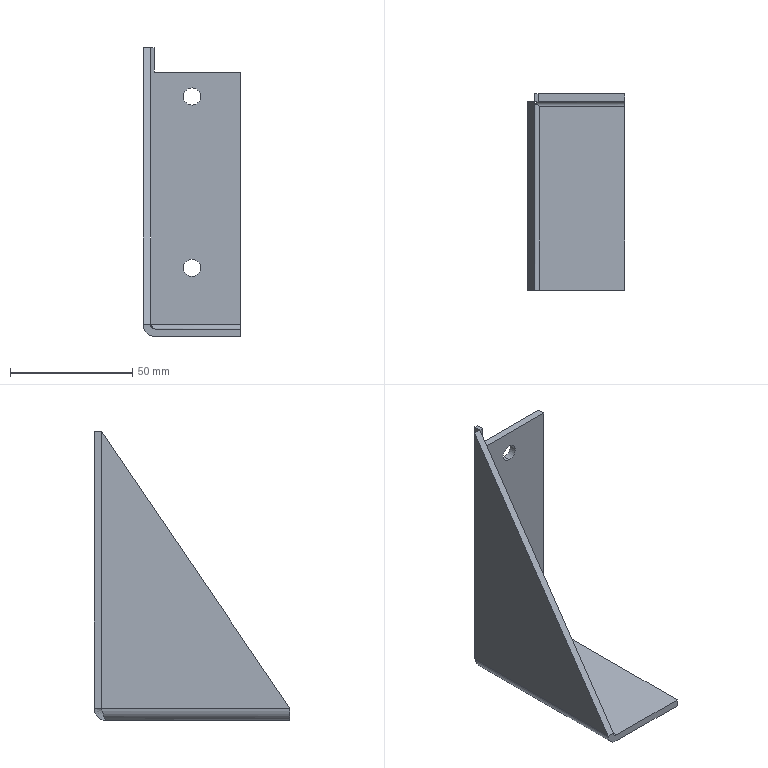Component | SolidWorks | ButtonStation-1_BracketAssembly-1_Bracket4-1 | 1 solid | 24 faces | box 40 x 80 x 118 mm | volume 33984 mm3 | plane 14 | cylinder 8 | spline 2 | commonest cylinder face diameters 7 x4 4 x2 10 x2 | material Plain Carbon Steel
STEP:
#1=COLOUR_RGB('',0.7922,0.8196,0.9333);
#2=FILL_AREA_STYLE_COLOUR('',#1);
#3=FILL_AREA_STYLE('',(#2));
#4=SURFACE_STYLE_FILL_AREA(#3);
#5=SURFACE_SIDE_STYLE('',(#4));
#6=SURFACE_STYLE_USAGE(.BOTH.,#5);
#7=PRESENTATION_STYLE_ASSIGNMENT((#6));
#8=CARTESIAN_POINT('',(-9.449,24.685,25.846));
#9=VERTEX_POINT('',#8);
#10=CARTESIAN_POINT('',(-9.449,24.685,25.571));
#11=VERTEX_POINT('',#10);
#12=CARTESIAN_POINT('',(-9.449,24.685,25.709));
#13=DIRECTION('',(0.,-1.,0.));
#14=DIRECTION('',(0.,0.,1.));
#15=AXIS2_PLACEMENT_3D('',#12,#13,#14);
#16=CIRCLE('',#15,0.1378);
#17=EDGE_CURVE('',#9,#11,#16,.T.);
#18=ORIENTED_EDGE('',*,*,#17,.T.);
#19=CARTESIAN_POINT('',(-9.449,24.803,25.571));
#20=VERTEX_POINT('',#19);
#21=CARTESIAN_POINT('',(-9.449,24.685,25.571));
#22=DIRECTION('',(0.,1.,-0.));
#23=VECTOR('',#22,39.37);
#24=LINE('',#21,#23);
#25=EDGE_CURVE('',#11,#20,#24,.T.);
#26=ORIENTED_EDGE('',*,*,#25,.T.);
#27=CARTESIAN_POINT('',(-9.449,24.803,25.846));
#28=VERTEX_POINT('',#27);
#29=CARTESIAN_POINT('',(-9.449,24.803,25.709));
#30=DIRECTION('',(0.,-1.,0.));
#31=DIRECTION('',(0.,0.,1.));
#32=AXIS2_PLACEMENT_3D('',#29,#30,#31);
#33=CIRCLE('',#32,0.1378);
#34=EDGE_CURVE('',#28,#20,#33,.T.);
#35=ORIENTED_EDGE('',*,*,#34,.F.);
#36=CARTESIAN_POINT('',(-9.449,24.685,25.846));
#37=DIRECTION('',(0.,1.,-0.));
#38=VECTOR('',#37,39.37);
#39=LINE('',#36,#38);
#40=EDGE_CURVE('',#9,#28,#39,.T.);
#41=ORIENTED_EDGE('',*,*,#40,.F.);
#42=EDGE_LOOP('',(#18,#26,#35,#41));
#43=FACE_OUTER_BOUND('',#42,.T.);
#44=CARTESIAN_POINT('',(-9.449,24.685,25.709));
#45=DIRECTION('',(0.,1.,-0.));
#46=DIRECTION('',(0.,0.,1.));
#47=AXIS2_PLACEMENT_3D('',#44,#45,#46);
#48=CYLINDRICAL_SURFACE('',#47,0.1378);
#49=ADVANCED_FACE('',(#43),#48,.F.);
#50=CARTESIAN_POINT('',(-9.449,24.685,23.091));
#51=VERTEX_POINT('',#50);
#52=CARTESIAN_POINT('',(-9.449,24.685,22.815));
#53=VERTEX_POINT('',#52);
#54=CARTESIAN_POINT('',(-9.449,24.685,22.953));
#55=DIRECTION('',(0.,-1.,0.));
#56=DIRECTION('',(0.,0.,1.));
#57=AXIS2_PLACEMENT_3D('',#54,#55,#56);
#58=CIRCLE('',#57,0.1378);
#59=EDGE_CURVE('',#51,#53,#58,.T.);
#60=ORIENTED_EDGE('',*,*,#59,.T.);
#61=CARTESIAN_POINT('',(-9.449,24.803,22.815));
#62=VERTEX_POINT('',#61);
#63=CARTESIAN_POINT('',(-9.449,24.685,22.815));
#64=DIRECTION('',(0.,1.,-0.));
#65=VECTOR('',#64,39.37);
#66=LINE('',#63,#65);
#67=EDGE_CURVE('',#53,#62,#66,.T.);
#68=ORIENTED_EDGE('',*,*,#67,.T.);
#69=CARTESIAN_POINT('',(-9.449,24.803,23.091));
#70=VERTEX_POINT('',#69);
#71=CARTESIAN_POINT('',(-9.449,24.803,22.953));
#72=DIRECTION('',(0.,-1.,0.));
#73=DIRECTION('',(0.,0.,1.));
#74=AXIS2_PLACEMENT_3D('',#71,#72,#73);
#75=CIRCLE('',#74,0.1378);
#76=EDGE_CURVE('',#70,#62,#75,.T.);
#77=ORIENTED_EDGE('',*,*,#76,.F.);
#78=CARTESIAN_POINT('',(-9.449,24.685,23.091));
#79=DIRECTION('',(0.,1.,-0.));
#80=VECTOR('',#79,39.37);
#81=LINE('',#78,#80);
#82=EDGE_CURVE('',#51,#70,#81,.T.);
#83=ORIENTED_EDGE('',*,*,#82,.F.);
#84=EDGE_LOOP('',(#60,#68,#77,#83));
#85=FACE_OUTER_BOUND('',#84,.T.);
#86=CARTESIAN_POINT('',(-9.449,24.685,22.953));
#87=DIRECTION('',(0.,1.,-0.));
#88=DIRECTION('',(0.,0.,1.));
#89=AXIS2_PLACEMENT_3D('',#86,#87,#88);
#90=CYLINDRICAL_SURFACE('',#89,0.1378);
#91=ADVANCED_FACE('',(#85),#90,.F.);
#92=CARTESIAN_POINT('',(-10.118,24.682,22.047));
#93=VERTEX_POINT('',#92);
#94=CARTESIAN_POINT('',(-10.118,21.654,22.047));
#95=VERTEX_POINT('',#94);
#96=CARTESIAN_POINT('',(-10.118,21.654,22.047));
#97=DIRECTION('',(0.,-1.,0.));
#98=VECTOR('',#97,39.37);
#99=LINE('',#96,#98);
#100=EDGE_CURVE('',#93,#95,#99,.T.);
#101=ORIENTED_EDGE('',*,*,#100,.F.);
#102=CARTESIAN_POINT('',(-10.118,24.682,26.496));
#103=VERTEX_POINT('',#102);
#104=CARTESIAN_POINT('',(-10.118,24.682,21.969));
#105=DIRECTION('',(0.,0.,-1.));
#106=VECTOR('',#105,39.37);
#107=LINE('',#104,#106);
#108=EDGE_CURVE('',#103,#93,#107,.T.);
#109=ORIENTED_EDGE('',*,*,#108,.F.);
#110=CARTESIAN_POINT('',(-10.118,21.654,22.047));
#111=DIRECTION('',(-0.,0.5628,0.8266));
#112=VECTOR('',#111,39.37);
#113=LINE('',#110,#112);
#114=EDGE_CURVE('',#95,#103,#113,.T.);
#115=ORIENTED_EDGE('',*,*,#114,.F.);
#116=EDGE_LOOP('',(#101,#109,#115));
#117=FACE_OUTER_BOUND('',#116,.T.);
#118=CARTESIAN_POINT('',(-10.118,21.654,21.969));
#119=DIRECTION('',(-1.,0.,-0.));
#120=DIRECTION('',(-0.,0.,1.));
#121=AXIS2_PLACEMENT_3D('',#118,#119,#120);
#122=PLANE('',#121);
#123=ADVANCED_FACE('',(#117),#122,.F.);
#124=CARTESIAN_POINT('',(-10.236,21.654,22.047));
#125=VERTEX_POINT('',#124);
#126=CARTESIAN_POINT('',(-10.236,21.654,22.047));
#127=DIRECTION('',(-1.,0.,-0.));
#128=VECTOR('',#127,39.37);
#129=LINE('',#126,#128);
#130=EDGE_CURVE('',#95,#125,#129,.T.);
#131=ORIENTED_EDGE('',*,*,#130,.F.);
#132=ORIENTED_EDGE('',*,*,#114,.T.);
#133=CARTESIAN_POINT('',(-10.236,24.682,26.496));
#134=VERTEX_POINT('',#133);
#135=CARTESIAN_POINT('',(-10.236,24.682,26.496));
#136=DIRECTION('',(1.,-0.,0.));
#137=VECTOR('',#136,39.37);
#138=LINE('',#135,#137);
#139=EDGE_CURVE('',#134,#103,#138,.T.);
#140=ORIENTED_EDGE('',*,*,#139,.F.);
#141=CARTESIAN_POINT('',(-10.236,24.682,26.496));
#142=DIRECTION('',(0.,0.5628,0.8266));
#143=VECTOR('',#142,39.37);
#144=LINE('',#141,#143);
#145=EDGE_CURVE('',#125,#134,#144,.T.);
#146=ORIENTED_EDGE('',*,*,#145,.F.);
#147=EDGE_LOOP('',(#131,#132,#140,#146));
#148=FACE_OUTER_BOUND('',#147,.T.);
#149=CARTESIAN_POINT('',(-10.236,24.682,26.496));
#150=DIRECTION('',(0.,0.8266,-0.5628));
#151=DIRECTION('',(0.,0.5628,0.8266));
#152=AXIS2_PLACEMENT_3D('',#149,#150,#151);
#153=PLANE('',#152);
#154=ADVANCED_FACE('',(#148),#153,.F.);
#155=CARTESIAN_POINT('',(-10.039,24.606,21.969));
#156=VERTEX_POINT('',#155);
#157=CARTESIAN_POINT('',(-10.118,24.682,22.047));
#158=CARTESIAN_POINT('',(-10.118,24.676,22.037));
#159=CARTESIAN_POINT('',(-10.116,24.67,22.027));
#160=CARTESIAN_POINT('',(-10.11,24.66,22.012));
#161=CARTESIAN_POINT('',(-10.108,24.657,22.008));
#162=CARTESIAN_POINT('',(-10.102,24.651,21.999));
#163=CARTESIAN_POINT('',(-10.099,24.648,21.995));
#164=CARTESIAN_POINT('',(-10.091,24.641,21.988));
#165=CARTESIAN_POINT('',(-10.087,24.638,21.985));
#166=CARTESIAN_POINT('',(-10.079,24.632,21.979));
#167=CARTESIAN_POINT('',(-10.074,24.629,21.977));
#168=CARTESIAN_POINT('',(-10.065,24.622,21.973));
#169=CARTESIAN_POINT('',(-10.06,24.619,21.971));
#170=CARTESIAN_POINT('',(-10.05,24.613,21.969));
#171=CARTESIAN_POINT('',(-10.045,24.609,21.969));
#172=CARTESIAN_POINT('',(-10.039,24.606,21.969));
#173=B_SPLINE_CURVE_WITH_KNOTS('',3,(#157,#158,#159,#160,#161,#162,#163,#164,#165,#166,#167,#168,#169,#170,#171,#172),.UNSPECIFIED.,.F.,.F.,(4,2,2,2,2,2,2,4),(0.,0.0009146,0.001372,0.001829,0.002286,0.002744,0.003201,0.003658),.UNSPECIFIED.);
#174=EDGE_CURVE('',#93,#156,#173,.T.);
#175=ORIENTED_EDGE('',*,*,#174,.F.);
#176=ORIENTED_EDGE('',*,*,#100,.T.);
#177=CARTESIAN_POINT('',(-10.039,21.654,21.969));
#178=VERTEX_POINT('',#177);
#179=CARTESIAN_POINT('',(-10.039,21.654,22.047));
#180=DIRECTION('',(0.,1.,0.));
#181=DIRECTION('',(0.,0.,-1.));
#182=AXIS2_PLACEMENT_3D('',#179,#180,#181);
#183=CIRCLE('',#182,0.07874);
#184=EDGE_CURVE('',#178,#95,#183,.T.);
#185=ORIENTED_EDGE('',*,*,#184,.F.);
#186=CARTESIAN_POINT('',(-10.039,21.654,21.969));
#187=DIRECTION('',(0.,-1.,0.));
#188=VECTOR('',#187,39.37);
#189=LINE('',#186,#188);
#190=EDGE_CURVE('',#156,#178,#189,.T.);
#191=ORIENTED_EDGE('',*,*,#190,.F.);
#192=EDGE_LOOP('',(#175,#176,#185,#191));
#193=FACE_OUTER_BOUND('',#192,.T.);
#194=CARTESIAN_POINT('',(-10.039,21.654,22.047));
#195=DIRECTION('',(0.,-1.,0.));
#196=DIRECTION('',(0.,0.,-1.));
#197=AXIS2_PLACEMENT_3D('',#194,#195,#196);
#198=CYLINDRICAL_SURFACE('',#197,0.07874);
#199=ADVANCED_FACE('',(#193),#198,.F.);
#200=CARTESIAN_POINT('',(-10.236,24.682,22.047));
#201=VERTEX_POINT('',#200);
#202=CARTESIAN_POINT('',(-10.118,24.682,22.047));
#203=DIRECTION('',(-1.,0.,0.));
#204=VECTOR('',#203,39.37);
#205=LINE('',#202,#204);
#206=EDGE_CURVE('',#93,#201,#205,.T.);
#207=ORIENTED_EDGE('',*,*,#206,.T.);
#208=CARTESIAN_POINT('',(-10.236,24.682,21.969));
#209=DIRECTION('',(0.,0.,1.));
#210=VECTOR('',#209,39.37);
#211=LINE('',#208,#210);
#212=EDGE_CURVE('',#201,#134,#211,.T.);
#213=ORIENTED_EDGE('',*,*,#212,.T.);
#214=ORIENTED_EDGE('',*,*,#139,.T.);
#215=ORIENTED_EDGE('',*,*,#108,.T.);
#216=EDGE_LOOP('',(#207,#213,#214,#215));
#217=FACE_OUTER_BOUND('',#216,.T.);
#218=CARTESIAN_POINT('',(-10.118,24.682,21.969));
#219=DIRECTION('',(0.,1.,0.));
#220=DIRECTION('',(0.,0.,1.));
#221=AXIS2_PLACEMENT_3D('',#218,#219,#220);
#222=PLANE('',#221);
#223=ADVANCED_FACE('',(#217),#222,.T.);
#224=ORIENTED_EDGE('',*,*,#145,.T.);
#225=ORIENTED_EDGE('',*,*,#212,.F.);
#226=CARTESIAN_POINT('',(-10.236,21.654,22.047));
#227=DIRECTION('',(0.,-1.,0.));
#228=VECTOR('',#227,39.37);
#229=LINE('',#226,#228);
#230=EDGE_CURVE('',#201,#125,#229,.T.);
#231=ORIENTED_EDGE('',*,*,#230,.T.);
#232=EDGE_LOOP('',(#224,#225,#231));
#233=FACE_OUTER_BOUND('',#232,.T.);
#234=CARTESIAN_POINT('',(-10.236,21.654,21.969));
#235=DIRECTION('',(-1.,0.,-0.));
#236=DIRECTION('',(-0.,0.,1.));
#237=AXIS2_PLACEMENT_3D('',#234,#235,#236);
#238=PLANE('',#237);
#239=ADVANCED_FACE('',(#233),#238,.T.);
#240=ORIENTED_EDGE('',*,*,#130,.T.);
#241=CARTESIAN_POINT('',(-10.039,21.654,21.85));
#242=VERTEX_POINT('',#241);
#243=CARTESIAN_POINT('',(-10.039,21.654,22.047));
#244=DIRECTION('',(0.,1.,0.));
#245=DIRECTION('',(0.,0.,-1.));
#246=AXIS2_PLACEMENT_3D('',#243,#244,#245);
#247=CIRCLE('',#246,0.1969);
#248=EDGE_CURVE('',#242,#125,#247,.T.);
#249=ORIENTED_EDGE('',*,*,#248,.F.);
#250=CARTESIAN_POINT('',(-8.661,21.654,21.85));
#251=VERTEX_POINT('',#250);
#252=CARTESIAN_POINT('',(-10.118,21.654,21.85));
#253=DIRECTION('',(-1.,0.,0.));
#254=VECTOR('',#253,39.37);
#255=LINE('',#252,#254);
#256=EDGE_CURVE('',#251,#242,#255,.T.);
#257=ORIENTED_EDGE('',*,*,#256,.F.);
#258=CARTESIAN_POINT('',(-8.661,21.654,21.969));
#259=VERTEX_POINT('',#258);
#260=CARTESIAN_POINT('',(-8.661,21.654,21.969));
#261=DIRECTION('',(0.,0.,-1.));
#262=VECTOR('',#261,39.37);
#263=LINE('',#260,#262);
#264=EDGE_CURVE('',#259,#251,#263,.T.);
#265=ORIENTED_EDGE('',*,*,#264,.F.);
#266=CARTESIAN_POINT('',(-10.118,21.654,21.969));
#267=DIRECTION('',(-1.,0.,0.));
#268=VECTOR('',#267,39.37);
#269=LINE('',#266,#268);
#270=EDGE_CURVE('',#259,#178,#269,.T.);
#271=ORIENTED_EDGE('',*,*,#270,.T.);
#272=ORIENTED_EDGE('',*,*,#184,.T.);
#273=EDGE_LOOP('',(#240,#249,#257,#265,#271,#272));
#274=FACE_OUTER_BOUND('',#273,.T.);
#275=CARTESIAN_POINT('',(-10.039,21.654,22.047));
#276=DIRECTION('',(0.,1.,0.));
#277=DIRECTION('',(0.,0.,1.));
#278=AXIS2_PLACEMENT_3D('',#275,#276,#277);
#279=PLANE('',#278);
#280=ADVANCED_FACE('',(#274),#279,.F.);
#281=ORIENTED_EDGE('',*,*,#190,.T.);
#282=ORIENTED_EDGE('',*,*,#270,.F.);
#283=CARTESIAN_POINT('',(-8.661,24.606,21.969));
#284=VERTEX_POINT('',#283);
#285=CARTESIAN_POINT('',(-8.661,24.685,21.969));
#286=DIRECTION('',(0.,-1.,0.));
#287=VECTOR('',#286,39.37);
#288=LINE('',#285,#287);
#289=EDGE_CURVE('',#284,#259,#288,.T.);
#290=ORIENTED_EDGE('',*,*,#289,.F.);
#291=CARTESIAN_POINT('',(-10.118,24.606,21.969));
#292=DIRECTION('',(1.,0.,0.));
#293=VECTOR('',#292,39.37);
#294=LINE('',#291,#293);
#295=EDGE_CURVE('',#156,#284,#294,.T.);
#296=ORIENTED_EDGE('',*,*,#295,.F.);
#297=EDGE_LOOP('',(#281,#282,#290,#296));
#298=FACE_OUTER_BOUND('',#297,.T.);
#299=CARTESIAN_POINT('',(-10.118,24.685,21.969));
#300=DIRECTION('',(0.,0.,-1.));
#301=DIRECTION('',(-1.,0.,0.));
#302=AXIS2_PLACEMENT_3D('',#299,#300,#301);
#303=PLANE('',#302);
#304=ADVANCED_FACE('',(#298),#303,.F.);
#305=ORIENTED_EDGE('',*,*,#174,.T.);
#306=CARTESIAN_POINT('',(-10.039,24.606,21.85));
#307=VERTEX_POINT('',#306);
#308=CARTESIAN_POINT('',(-10.039,24.606,21.909));
#309=DIRECTION('',(0.,0.,1.));
#310=VECTOR('',#309,39.37);
#311=LINE('',#308,#310);
#312=EDGE_CURVE('',#307,#156,#311,.T.);
#313=ORIENTED_EDGE('',*,*,#312,.F.);
#314=CARTESIAN_POINT('',(-10.236,24.682,22.047));
#315=CARTESIAN_POINT('',(-10.236,24.679,22.034));
#316=CARTESIAN_POINT('',(-10.235,24.676,22.021));
#317=CARTESIAN_POINT('',(-10.23,24.67,21.996));
#318=CARTESIAN_POINT('',(-10.226,24.666,21.984));
#319=CARTESIAN_POINT('',(-10.216,24.66,21.96));
#320=CARTESIAN_POINT('',(-10.21,24.657,21.949));
#321=CARTESIAN_POINT('',(-10.196,24.651,21.927));
#322=CARTESIAN_POINT('',(-10.188,24.647,21.917));
#323=CARTESIAN_POINT('',(-10.17,24.641,21.899));
#324=CARTESIAN_POINT('',(-10.16,24.638,21.891));
#325=CARTESIAN_POINT('',(-10.138,24.632,21.876));
#326=CARTESIAN_POINT('',(-10.127,24.628,21.87));
#327=CARTESIAN_POINT('',(-10.103,24.622,21.861));
#328=CARTESIAN_POINT('',(-10.091,24.619,21.857));
#329=CARTESIAN_POINT('',(-10.065,24.613,21.852));
#330=CARTESIAN_POINT('',(-10.052,24.609,21.85));
#331=CARTESIAN_POINT('',(-10.039,24.606,21.85));
#332=B_SPLINE_CURVE_WITH_KNOTS('',3,(#314,#315,#316,#317,#318,#319,#320,#321,#322,#323,#324,#325,#326,#327,#328,#329,#330,#331),.UNSPECIFIED.,.F.,.F.,(4,2,2,2,2,2,2,2,4),(0.,0.001008,0.002017,0.003025,0.004033,0.005041,0.00605,0.007058,0.008066),.UNSPECIFIED.);
#333=EDGE_CURVE('',#201,#307,#332,.T.);
#334=ORIENTED_EDGE('',*,*,#333,.F.);
#335=ORIENTED_EDGE('',*,*,#206,.F.);
#336=EDGE_LOOP('',(#305,#313,#334,#335));
#337=FACE_OUTER_BOUND('',#336,.T.);
#338=CARTESIAN_POINT('',(-10.039,24.606,21.849));
#339=CARTESIAN_POINT('',(-10.065,24.613,21.849));
#340=CARTESIAN_POINT('',(-10.091,24.619,21.854));
#341=CARTESIAN_POINT('',(-10.139,24.632,21.874));
#342=CARTESIAN_POINT('',(-10.161,24.638,21.889));
#343=CARTESIAN_POINT('',(-10.198,24.651,21.926));
#344=CARTESIAN_POINT('',(-10.212,24.657,21.948));
#345=CARTESIAN_POINT('',(-10.232,24.67,21.995));
#346=CARTESIAN_POINT('',(-10.237,24.676,22.021));
#347=CARTESIAN_POINT('',(-10.237,24.682,22.047));
#348=CARTESIAN_POINT('',(-10.039,24.606,21.85));
#349=CARTESIAN_POINT('',(-10.065,24.613,21.85));
#350=CARTESIAN_POINT('',(-10.091,24.619,21.856));
#351=CARTESIAN_POINT('',(-10.139,24.632,21.875));
#352=CARTESIAN_POINT('',(-10.16,24.638,21.89));
#353=CARTESIAN_POINT('',(-10.197,24.651,21.926));
#354=CARTESIAN_POINT('',(-10.211,24.657,21.948));
#355=CARTESIAN_POINT('',(-10.231,24.67,21.996));
#356=CARTESIAN_POINT('',(-10.236,24.676,22.021));
#357=CARTESIAN_POINT('',(-10.236,24.682,22.047));
#358=CARTESIAN_POINT('',(-10.039,24.606,21.969));
#359=CARTESIAN_POINT('',(-10.05,24.613,21.969));
#360=CARTESIAN_POINT('',(-10.06,24.619,21.971));
#361=CARTESIAN_POINT('',(-10.079,24.632,21.978));
#362=CARTESIAN_POINT('',(-10.088,24.638,21.984));
#363=CARTESIAN_POINT('',(-10.102,24.651,21.999));
#364=CARTESIAN_POINT('',(-10.108,24.657,22.008));
#365=CARTESIAN_POINT('',(-10.116,24.67,22.027));
#366=CARTESIAN_POINT('',(-10.118,24.676,22.037));
#367=CARTESIAN_POINT('',(-10.118,24.682,22.047));
#368=CARTESIAN_POINT('',(-10.039,24.606,21.97));
#369=CARTESIAN_POINT('',(-10.05,24.613,21.97));
#370=CARTESIAN_POINT('',(-10.06,24.619,21.972));
#371=CARTESIAN_POINT('',(-10.078,24.632,21.979));
#372=CARTESIAN_POINT('',(-10.087,24.638,21.985));
#373=CARTESIAN_POINT('',(-10.101,24.651,22.));
#374=CARTESIAN_POINT('',(-10.107,24.657,22.008));
#375=CARTESIAN_POINT('',(-10.115,24.67,22.027));
#376=CARTESIAN_POINT('',(-10.117,24.676,22.037));
#377=CARTESIAN_POINT('',(-10.117,24.682,22.047));
#378=B_SPLINE_SURFACE_WITH_KNOTS('',1,3,((#338,#339,#340,#341,#342,#343,#344,#345,#346,#347),(#348,#349,#350,#351,#352,#353,#354,#355,#356,#357),(#358,#359,#360,#361,#362,#363,#364,#365,#366,#367),(#368,#369,#370,#371,#372,#373,#374,#375,#376,#377)),.UNSPECIFIED.,.F.,.F.,.F.,(2,1,1,2),(4,2,2,2,4),(-0.01,0.,1.,1.01),(0.,0.25,0.5,0.75,1.),.UNSPECIFIED.);
#379=ADVANCED_FACE('',(#337),#378,.F.);
#380=ORIENTED_EDGE('',*,*,#230,.F.);
#381=ORIENTED_EDGE('',*,*,#333,.T.);
#382=CARTESIAN_POINT('',(-10.039,21.654,21.85));
#383=DIRECTION('',(0.,-1.,0.));
#384=VECTOR('',#383,39.37);
#385=LINE('',#382,#384);
#386=EDGE_CURVE('',#307,#242,#385,.T.);
#387=ORIENTED_EDGE('',*,*,#386,.T.);
#388=ORIENTED_EDGE('',*,*,#248,.T.);
#389=EDGE_LOOP('',(#380,#381,#387,#388));
#390=FACE_OUTER_BOUND('',#389,.T.);
#391=CARTESIAN_POINT('',(-10.039,21.654,22.047));
#392=DIRECTION('',(0.,-1.,0.));
#393=DIRECTION('',(0.,0.,-1.));
#394=AXIS2_PLACEMENT_3D('',#391,#392,#393);
#395=CYLINDRICAL_SURFACE('',#394,0.1969);
#396=ADVANCED_FACE('',(#390),#395,.T.);
#397=CARTESIAN_POINT('',(-8.661,24.685,22.047));
#398=VERTEX_POINT('',#397);
#399=CARTESIAN_POINT('',(-8.661,24.606,22.047));
#400=DIRECTION('',(-1.,0.,0.));
#401=DIRECTION('',(0.,0.,1.));
#402=AXIS2_PLACEMENT_3D('',#399,#400,#401);
#403=CIRCLE('',#402,0.07874);
#404=EDGE_CURVE('',#398,#284,#403,.T.);
#405=ORIENTED_EDGE('',*,*,#404,.F.);
#406=CARTESIAN_POINT('',(-10.115,24.685,22.047));
#407=VERTEX_POINT('',#406);
#408=CARTESIAN_POINT('',(-10.115,24.685,22.047));
#409=DIRECTION('',(1.,0.,0.));
#410=VECTOR('',#409,39.37);
#411=LINE('',#408,#410);
#412=EDGE_CURVE('',#407,#398,#411,.T.);
#413=ORIENTED_EDGE('',*,*,#412,.F.);
#414=CARTESIAN_POINT('',(-10.039,24.606,21.969));
#415=CARTESIAN_POINT('',(-10.046,24.617,21.969));
#416=CARTESIAN_POINT('',(-10.052,24.627,21.971));
#417=CARTESIAN_POINT('',(-10.061,24.641,21.976));
#418=CARTESIAN_POINT('',(-10.065,24.646,21.979));
#419=CARTESIAN_POINT('',(-10.071,24.654,21.985));
#420=CARTESIAN_POINT('',(-10.074,24.658,21.988));
#421=CARTESIAN_POINT('',(-10.08,24.666,21.995));
#422=CARTESIAN_POINT('',(-10.084,24.669,21.999));
#423=CARTESIAN_POINT('',(-10.09,24.675,22.008));
#424=CARTESIAN_POINT('',(-10.093,24.677,22.012));
#425=CARTESIAN_POINT('',(-10.099,24.681,22.022));
#426=CARTESIAN_POINT('',(-10.103,24.683,22.027));
#427=CARTESIAN_POINT('',(-10.109,24.685,22.037));
#428=CARTESIAN_POINT('',(-10.112,24.685,22.042));
#429=CARTESIAN_POINT('',(-10.115,24.685,22.047));
#430=B_SPLINE_CURVE_WITH_KNOTS('',3,(#414,#415,#416,#417,#418,#419,#420,#421,#422,#423,#424,#425,#426,#427,#428,#429),.UNSPECIFIED.,.F.,.F.,(4,2,2,2,2,2,2,4),(0.,0.0009146,0.001372,0.001829,0.002286,0.002744,0.003201,0.003658),.UNSPECIFIED.);
#431=EDGE_CURVE('',#156,#407,#430,.T.);
#432=ORIENTED_EDGE('',*,*,#431,.F.);
#433=ORIENTED_EDGE('',*,*,#295,.T.);
#434=EDGE_LOOP('',(#405,#413,#432,#433));
#435=FACE_OUTER_BOUND('',#434,.T.);
#436=CARTESIAN_POINT('',(-10.115,24.606,22.047));
#437=DIRECTION('',(-1.,0.,0.));
#438=DIRECTION('',(0.,0.,1.));
#439=AXIS2_PLACEMENT_3D('',#436,#437,#438);
#440=CYLINDRICAL_SURFACE('',#439,0.07874);
#441=ADVANCED_FACE('',(#435),#440,.F.);
#442=CARTESIAN_POINT('',(-8.661,24.803,22.047));
#443=VERTEX_POINT('',#442);
#444=CARTESIAN_POINT('',(-8.661,24.803,26.102));
#445=VERTEX_POINT('',#444);
#446=CARTESIAN_POINT('',(-8.661,24.803,26.496));
#447=DIRECTION('',(0.,0.,1.));
#448=VECTOR('',#447,39.37);
#449=LINE('',#446,#448);
#450=EDGE_CURVE('',#443,#445,#449,.T.);
#451=ORIENTED_EDGE('',*,*,#450,.T.);
#452=CARTESIAN_POINT('',(-8.661,24.685,26.102));
#453=VERTEX_POINT('',#452);
#454=CARTESIAN_POINT('',(-8.661,21.654,26.102));
#455=DIRECTION('',(0.,-1.,0.));
#456=VECTOR('',#455,39.37);
#457=LINE('',#454,#456);
#458=EDGE_CURVE('',#445,#453,#457,.T.);
#459=ORIENTED_EDGE('',*,*,#458,.T.);
#460=CARTESIAN_POINT('',(-8.661,24.685,21.969));
#461=DIRECTION('',(0.,-0.,-1.));
#462=VECTOR('',#461,39.37);
#463=LINE('',#460,#462);
#464=EDGE_CURVE('',#453,#398,#463,.T.);
#465=ORIENTED_EDGE('',*,*,#464,.T.);
#466=ORIENTED_EDGE('',*,*,#404,.T.);
#467=ORIENTED_EDGE('',*,*,#289,.T.);
#468=ORIENTED_EDGE('',*,*,#264,.T.);
#469=CARTESIAN_POINT('',(-8.661,24.606,21.85));
#470=VERTEX_POINT('',#469);
#471=CARTESIAN_POINT('',(-8.661,21.654,21.85));
#472=DIRECTION('',(0.,-1.,0.));
#473=VECTOR('',#472,39.37);
#474=LINE('',#471,#473);
#475=EDGE_CURVE('',#470,#251,#474,.T.);
#476=ORIENTED_EDGE('',*,*,#475,.F.);
#477=CARTESIAN_POINT('',(-8.661,24.606,22.047));
#478=DIRECTION('',(1.,0.,0.));
#479=DIRECTION('',(0.,0.,1.));
#480=AXIS2_PLACEMENT_3D('',#477,#478,#479);
#481=CIRCLE('',#480,0.1969);
#482=EDGE_CURVE('',#470,#443,#481,.T.);
#483=ORIENTED_EDGE('',*,*,#482,.T.);
#484=EDGE_LOOP('',(#451,#459,#465,#466,#467,#468,#476,#483));
#485=FACE_OUTER_BOUND('',#484,.T.);
#486=CARTESIAN_POINT('',(-8.661,21.654,21.969));
#487=DIRECTION('',(-1.,0.,0.));
#488=DIRECTION('',(0.,0.,1.));
#489=AXIS2_PLACEMENT_3D('',#486,#487,#488);
#490=PLANE('',#489);
#491=ADVANCED_FACE('',(#485),#490,.F.);
#492=CARTESIAN_POINT('',(-10.115,24.803,22.047));
#493=VERTEX_POINT('',#492);
#494=CARTESIAN_POINT('',(-10.115,24.744,22.047));
#495=DIRECTION('',(0.,-1.,0.));
#496=VECTOR('',#495,39.37);
#497=LINE('',#494,#496);
#498=EDGE_CURVE('',#493,#407,#497,.T.);
#499=ORIENTED_EDGE('',*,*,#498,.F.);
#500=CARTESIAN_POINT('',(-10.039,24.606,21.85));
#501=CARTESIAN_POINT('',(-10.043,24.619,21.85));
#502=CARTESIAN_POINT('',(-10.046,24.632,21.852));
#503=CARTESIAN_POINT('',(-10.052,24.657,21.857));
#504=CARTESIAN_POINT('',(-10.055,24.67,21.86));
#505=CARTESIAN_POINT('',(-10.062,24.694,21.87));
#506=CARTESIAN_POINT('',(-10.065,24.705,21.876));
#507=CARTESIAN_POINT('',(-10.071,24.726,21.891));
#508=CARTESIAN_POINT('',(-10.074,24.736,21.899));
#509=CARTESIAN_POINT('',(-10.08,24.755,21.917));
#510=CARTESIAN_POINT('',(-10.084,24.763,21.927));
#511=CARTESIAN_POINT('',(-10.09,24.777,21.949));
#512=CARTESIAN_POINT('',(-10.093,24.783,21.96));
#513=CARTESIAN_POINT('',(-10.099,24.793,21.984));
#514=CARTESIAN_POINT('',(-10.103,24.797,21.996));
#515=CARTESIAN_POINT('',(-10.109,24.802,22.021));
#516=CARTESIAN_POINT('',(-10.112,24.803,22.034));
#517=CARTESIAN_POINT('',(-10.115,24.803,22.047));
#518=B_SPLINE_CURVE_WITH_KNOTS('',3,(#500,#501,#502,#503,#504,#505,#506,#507,#508,#509,#510,#511,#512,#513,#514,#515,#516,#517),.UNSPECIFIED.,.F.,.F.,(4,2,2,2,2,2,2,2,4),(0.,0.001008,0.002017,0.003025,0.004033,0.005041,0.00605,0.007058,0.008066),.UNSPECIFIED.);
#519=EDGE_CURVE('',#307,#493,#518,.T.);
#520=ORIENTED_EDGE('',*,*,#519,.F.);
#521=ORIENTED_EDGE('',*,*,#312,.T.);
#522=ORIENTED_EDGE('',*,*,#431,.T.);
#523=EDGE_LOOP('',(#499,#520,#521,#522));
#524=FACE_OUTER_BOUND('',#523,.T.);
#525=CARTESIAN_POINT('',(-10.115,24.804,22.047));
#526=CARTESIAN_POINT('',(-10.109,24.804,22.021));
#527=CARTESIAN_POINT('',(-10.103,24.799,21.995));
#528=CARTESIAN_POINT('',(-10.09,24.779,21.948));
#529=CARTESIAN_POINT('',(-10.084,24.765,21.926));
#530=CARTESIAN_POINT('',(-10.071,24.728,21.889));
#531=CARTESIAN_POINT('',(-10.065,24.706,21.874));
#532=CARTESIAN_POINT('',(-10.052,24.658,21.854));
#533=CARTESIAN_POINT('',(-10.046,24.632,21.849));
#534=CARTESIAN_POINT('',(-10.039,24.606,21.849));
#535=CARTESIAN_POINT('',(-10.115,24.803,22.047));
#536=CARTESIAN_POINT('',(-10.109,24.803,22.021));
#537=CARTESIAN_POINT('',(-10.103,24.798,21.996));
#538=CARTESIAN_POINT('',(-10.09,24.778,21.948));
#539=CARTESIAN_POINT('',(-10.084,24.764,21.926));
#540=CARTESIAN_POINT('',(-10.071,24.727,21.89));
#541=CARTESIAN_POINT('',(-10.065,24.705,21.875));
#542=CARTESIAN_POINT('',(-10.052,24.658,21.856));
#543=CARTESIAN_POINT('',(-10.046,24.632,21.85));
#544=CARTESIAN_POINT('',(-10.039,24.606,21.85));
#545=CARTESIAN_POINT('',(-10.115,24.685,22.047));
#546=CARTESIAN_POINT('',(-10.109,24.685,22.037));
#547=CARTESIAN_POINT('',(-10.103,24.683,22.027));
#548=CARTESIAN_POINT('',(-10.09,24.675,22.008));
#549=CARTESIAN_POINT('',(-10.084,24.669,21.999));
#550=CARTESIAN_POINT('',(-10.071,24.655,21.984));
#551=CARTESIAN_POINT('',(-10.065,24.646,21.978));
#552=CARTESIAN_POINT('',(-10.052,24.627,21.971));
#553=CARTESIAN_POINT('',(-10.046,24.617,21.969));
#554=CARTESIAN_POINT('',(-10.039,24.606,21.969));
#555=CARTESIAN_POINT('',(-10.115,24.684,22.047));
#556=CARTESIAN_POINT('',(-10.109,24.684,22.037));
#557=CARTESIAN_POINT('',(-10.103,24.682,22.027));
#558=CARTESIAN_POINT('',(-10.09,24.674,22.008));
#559=CARTESIAN_POINT('',(-10.084,24.668,22.));
#560=CARTESIAN_POINT('',(-10.071,24.654,21.985));
#561=CARTESIAN_POINT('',(-10.065,24.645,21.979));
#562=CARTESIAN_POINT('',(-10.052,24.627,21.972));
#563=CARTESIAN_POINT('',(-10.046,24.616,21.97));
#564=CARTESIAN_POINT('',(-10.039,24.606,21.97));
#565=B_SPLINE_SURFACE_WITH_KNOTS('',1,3,((#525,#526,#527,#528,#529,#530,#531,#532,#533,#534),(#535,#536,#537,#538,#539,#540,#541,#542,#543,#544),(#545,#546,#547,#548,#549,#550,#551,#552,#553,#554),(#555,#556,#557,#558,#559,#560,#561,#562,#563,#564)),.UNSPECIFIED.,.F.,.F.,.F.,(2,1,1,2),(4,2,2,2,4),(-0.01,0.,1.,1.01),(0.,0.25,0.5,0.75,1.),.UNSPECIFIED.);
#566=ADVANCED_FACE('',(#524),#565,.F.);
#567=ORIENTED_EDGE('',*,*,#475,.T.);
#568=ORIENTED_EDGE('',*,*,#256,.T.);
#569=ORIENTED_EDGE('',*,*,#386,.F.);
#570=CARTESIAN_POINT('',(-10.118,24.606,21.85));
#571=DIRECTION('',(1.,0.,0.));
#572=VECTOR('',#571,39.37);
#573=LINE('',#570,#572);
#574=EDGE_CURVE('',#307,#470,#573,.T.);
#575=ORIENTED_EDGE('',*,*,#574,.T.);
#576=EDGE_LOOP('',(#567,#568,#569,#575));
#577=FACE_OUTER_BOUND('',#576,.T.);
#578=CARTESIAN_POINT('',(-10.118,24.685,21.85));
#579=DIRECTION('',(0.,0.,-1.));
#580=DIRECTION('',(-1.,0.,0.));
#581=AXIS2_PLACEMENT_3D('',#578,#579,#580);
#582=PLANE('',#581);
#583=ADVANCED_FACE('',(#577),#582,.T.);
#584=CARTESIAN_POINT('',(-10.059,24.685,26.102));
#585=VERTEX_POINT('',#584);
#586=CARTESIAN_POINT('',(-10.118,24.685,26.102));
#587=DIRECTION('',(-1.,0.,0.));
#588=VECTOR('',#587,39.37);
#589=LINE('',#586,#588);
#590=EDGE_CURVE('',#453,#585,#589,.T.);
#591=ORIENTED_EDGE('',*,*,#590,.T.);
#592=CARTESIAN_POINT('',(-10.059,24.685,26.496));
#593=VERTEX_POINT('',#592);
#594=CARTESIAN_POINT('',(-10.059,24.685,21.969));
#595=DIRECTION('',(0.,0.,1.));
#596=VECTOR('',#595,39.37);
#597=LINE('',#594,#596);
#598=EDGE_CURVE('',#585,#593,#597,.T.);
#599=ORIENTED_EDGE('',*,*,#598,.T.);
#600=CARTESIAN_POINT('',(-10.115,24.685,26.496));
#601=VERTEX_POINT('',#600);
#602=CARTESIAN_POINT('',(-10.118,24.685,26.496));
#603=DIRECTION('',(1.,0.,0.));
#604=VECTOR('',#603,39.37);
#605=LINE('',#602,#604);
#606=EDGE_CURVE('',#601,#593,#605,.T.);
#607=ORIENTED_EDGE('',*,*,#606,.F.);
#608=CARTESIAN_POINT('',(-10.115,24.685,21.969));
#609=DIRECTION('',(0.,0.,1.));
#610=VECTOR('',#609,39.37);
#611=LINE('',#608,#610);
#612=EDGE_CURVE('',#407,#601,#611,.T.);
#613=ORIENTED_EDGE('',*,*,#612,.F.);
#614=ORIENTED_EDGE('',*,*,#412,.T.);
#615=ORIENTED_EDGE('',*,*,#464,.F.);
#616=EDGE_LOOP('',(#591,#599,#607,#613,#614,#615));
#617=FACE_OUTER_BOUND('',#616,.T.);
#618=ORIENTED_EDGE('',*,*,#17,.F.);
#619=CARTESIAN_POINT('',(-9.449,24.685,25.709));
#620=DIRECTION('',(0.,-1.,0.));
#621=DIRECTION('',(0.,0.,1.));
#622=AXIS2_PLACEMENT_3D('',#619,#620,#621);
#623=CIRCLE('',#622,0.1378);
#624=EDGE_CURVE('',#11,#9,#623,.T.);
#625=ORIENTED_EDGE('',*,*,#624,.F.);
#626=EDGE_LOOP('',(#618,#625));
#627=FACE_BOUND('',#626,.T.);
#628=ORIENTED_EDGE('',*,*,#59,.F.);
#629=CARTESIAN_POINT('',(-9.449,24.685,22.953));
#630=DIRECTION('',(0.,-1.,0.));
#631=DIRECTION('',(0.,0.,1.));
#632=AXIS2_PLACEMENT_3D('',#629,#630,#631);
#633=CIRCLE('',#632,0.1378);
#634=EDGE_CURVE('',#53,#51,#633,.T.);
#635=ORIENTED_EDGE('',*,*,#634,.F.);
#636=EDGE_LOOP('',(#628,#635));
#637=FACE_BOUND('',#636,.T.);
#638=CARTESIAN_POINT('',(-10.118,24.685,21.969));
#639=DIRECTION('',(0.,1.,-0.));
#640=DIRECTION('',(0.,0.,1.));
#641=AXIS2_PLACEMENT_3D('',#638,#639,#640);
#642=PLANE('',#641);
#643=ADVANCED_FACE('',(#617,#627,#637),#642,.F.);
#644=CARTESIAN_POINT('',(-10.115,24.803,26.496));
#645=VERTEX_POINT('',#644);
#646=CARTESIAN_POINT('',(-10.115,24.685,26.496));
#647=DIRECTION('',(0.,-1.,0.));
#648=VECTOR('',#647,39.37);
#649=LINE('',#646,#648);
#650=EDGE_CURVE('',#645,#601,#649,.T.);
#651=ORIENTED_EDGE('',*,*,#650,.F.);
#652=CARTESIAN_POINT('',(-10.115,24.803,21.969));
#653=DIRECTION('',(0.,0.,1.));
#654=VECTOR('',#653,39.37);
#655=LINE('',#652,#654);
#656=EDGE_CURVE('',#493,#645,#655,.T.);
#657=ORIENTED_EDGE('',*,*,#656,.F.);
#658=ORIENTED_EDGE('',*,*,#498,.T.);
#659=ORIENTED_EDGE('',*,*,#612,.T.);
#660=EDGE_LOOP('',(#651,#657,#658,#659));
#661=FACE_OUTER_BOUND('',#660,.T.);
#662=CARTESIAN_POINT('',(-10.115,24.685,21.969));
#663=DIRECTION('',(1.,0.,0.));
#664=DIRECTION('',(0.,0.,-1.));
#665=AXIS2_PLACEMENT_3D('',#662,#663,#664);
#666=PLANE('',#665);
#667=ADVANCED_FACE('',(#661),#666,.F.);
#668=CARTESIAN_POINT('',(-10.115,24.803,22.047));
#669=DIRECTION('',(1.,0.,0.));
#670=VECTOR('',#669,39.37);
#671=LINE('',#668,#670);
#672=EDGE_CURVE('',#493,#443,#671,.T.);
#673=ORIENTED_EDGE('',*,*,#672,.T.);
#674=ORIENTED_EDGE('',*,*,#482,.F.);
#675=ORIENTED_EDGE('',*,*,#574,.F.);
#676=ORIENTED_EDGE('',*,*,#519,.T.);
#677=EDGE_LOOP('',(#673,#674,#675,#676));
#678=FACE_OUTER_BOUND('',#677,.T.);
#679=CARTESIAN_POINT('',(-10.115,24.606,22.047));
#680=DIRECTION('',(-1.,0.,0.));
#681=DIRECTION('',(0.,0.,1.));
#682=AXIS2_PLACEMENT_3D('',#679,#680,#681);
#683=CYLINDRICAL_SURFACE('',#682,0.1969);
#684=ADVANCED_FACE('',(#678),#683,.T.);
#685=CARTESIAN_POINT('',(-10.059,24.803,26.496));
#686=VERTEX_POINT('',#685);
#687=CARTESIAN_POINT('',(-10.059,24.803,26.496));
#688=DIRECTION('',(0.,-1.,0.));
#689=VECTOR('',#688,39.37);
#690=LINE('',#687,#689);
#691=EDGE_CURVE('',#686,#593,#690,.T.);
#692=ORIENTED_EDGE('',*,*,#691,.F.);
#693=CARTESIAN_POINT('',(-10.118,24.803,26.496));
#694=DIRECTION('',(-1.,0.,0.));
#695=VECTOR('',#694,39.37);
#696=LINE('',#693,#695);
#697=EDGE_CURVE('',#686,#645,#696,.T.);
#698=ORIENTED_EDGE('',*,*,#697,.T.);
#699=ORIENTED_EDGE('',*,*,#650,.T.);
#700=ORIENTED_EDGE('',*,*,#606,.T.);
#701=EDGE_LOOP('',(#692,#698,#699,#700));
#702=FACE_OUTER_BOUND('',#701,.T.);
#703=CARTESIAN_POINT('',(-10.118,24.803,26.496));
#704=DIRECTION('',(0.,0.,1.));
#705=DIRECTION('',(0.,-1.,0.));
#706=AXIS2_PLACEMENT_3D('',#703,#704,#705);
#707=PLANE('',#706);
#708=ADVANCED_FACE('',(#702),#707,.T.);
#709=ORIENTED_EDGE('',*,*,#25,.F.);
#710=ORIENTED_EDGE('',*,*,#624,.T.);
#711=ORIENTED_EDGE('',*,*,#40,.T.);
#712=CARTESIAN_POINT('',(-9.449,24.803,25.709));
#713=DIRECTION('',(0.,-1.,0.));
#714=DIRECTION('',(0.,0.,1.));
#715=AXIS2_PLACEMENT_3D('',#712,#713,#714);
#716=CIRCLE('',#715,0.1378);
#717=EDGE_CURVE('',#20,#28,#716,.T.);
#718=ORIENTED_EDGE('',*,*,#717,.F.);
#719=EDGE_LOOP('',(#709,#710,#711,#718));
#720=FACE_OUTER_BOUND('',#719,.T.);
#721=CARTESIAN_POINT('',(-9.449,24.685,25.709));
#722=DIRECTION('',(0.,1.,-0.));
#723=DIRECTION('',(0.,0.,1.));
#724=AXIS2_PLACEMENT_3D('',#721,#722,#723);
#725=CYLINDRICAL_SURFACE('',#724,0.1378);
#726=ADVANCED_FACE('',(#720),#725,.F.);
#727=ORIENTED_EDGE('',*,*,#67,.F.);
#728=ORIENTED_EDGE('',*,*,#634,.T.);
#729=ORIENTED_EDGE('',*,*,#82,.T.);
#730=CARTESIAN_POINT('',(-9.449,24.803,22.953));
#731=DIRECTION('',(0.,-1.,0.));
#732=DIRECTION('',(0.,0.,1.));
#733=AXIS2_PLACEMENT_3D('',#730,#731,#732);
#734=CIRCLE('',#733,0.1378);
#735=EDGE_CURVE('',#62,#70,#734,.T.);
#736=ORIENTED_EDGE('',*,*,#735,.F.);
#737=EDGE_LOOP('',(#727,#728,#729,#736));
#738=FACE_OUTER_BOUND('',#737,.T.);
#739=CARTESIAN_POINT('',(-9.449,24.685,22.953));
#740=DIRECTION('',(0.,1.,-0.));
#741=DIRECTION('',(0.,0.,1.));
#742=AXIS2_PLACEMENT_3D('',#739,#740,#741);
#743=CYLINDRICAL_SURFACE('',#742,0.1378);
#744=ADVANCED_FACE('',(#738),#743,.F.);
#745=CARTESIAN_POINT('',(-10.059,24.803,26.102));
#746=VERTEX_POINT('',#745);
#747=CARTESIAN_POINT('',(-10.059,24.803,21.969));
#748=DIRECTION('',(0.,0.,1.));
#749=VECTOR('',#748,39.37);
#750=LINE('',#747,#749);
#751=EDGE_CURVE('',#746,#686,#750,.T.);
#752=ORIENTED_EDGE('',*,*,#751,.F.);
#753=CARTESIAN_POINT('',(-10.118,24.803,26.102));
#754=DIRECTION('',(-1.,0.,0.));
#755=VECTOR('',#754,39.37);
#756=LINE('',#753,#755);
#757=EDGE_CURVE('',#445,#746,#756,.T.);
#758=ORIENTED_EDGE('',*,*,#757,.F.);
#759=ORIENTED_EDGE('',*,*,#450,.F.);
#760=ORIENTED_EDGE('',*,*,#672,.F.);
#761=ORIENTED_EDGE('',*,*,#656,.T.);
#762=ORIENTED_EDGE('',*,*,#697,.F.);
#763=EDGE_LOOP('',(#752,#758,#759,#760,#761,#762));
#764=FACE_OUTER_BOUND('',#763,.T.);
#765=ORIENTED_EDGE('',*,*,#34,.T.);
#766=ORIENTED_EDGE('',*,*,#717,.T.);
#767=EDGE_LOOP('',(#765,#766));
#768=FACE_BOUND('',#767,.T.);
#769=ORIENTED_EDGE('',*,*,#76,.T.);
#770=ORIENTED_EDGE('',*,*,#735,.T.);
#771=EDGE_LOOP('',(#769,#770));
#772=FACE_BOUND('',#771,.T.);
#773=CARTESIAN_POINT('',(-10.118,24.803,21.969));
#774=DIRECTION('',(0.,1.,-0.));
#775=DIRECTION('',(0.,0.,1.));
#776=AXIS2_PLACEMENT_3D('',#773,#774,#775);
#777=PLANE('',#776);
#778=ADVANCED_FACE('',(#764,#768,#772),#777,.T.);
#779=ORIENTED_EDGE('',*,*,#458,.F.);
#780=ORIENTED_EDGE('',*,*,#757,.T.);
#781=CARTESIAN_POINT('',(-10.059,21.654,26.102));
#782=DIRECTION('',(0.,1.,0.));
#783=VECTOR('',#782,39.37);
#784=LINE('',#781,#783);
#785=EDGE_CURVE('',#585,#746,#784,.T.);
#786=ORIENTED_EDGE('',*,*,#785,.F.);
#787=ORIENTED_EDGE('',*,*,#590,.F.);
#788=EDGE_LOOP('',(#779,#780,#786,#787));
#789=FACE_OUTER_BOUND('',#788,.T.);
#790=CARTESIAN_POINT('',(-10.059,21.654,26.102));
#791=DIRECTION('',(0.,0.,-1.));
#792=DIRECTION('',(-1.,0.,0.));
#793=AXIS2_PLACEMENT_3D('',#790,#791,#792);
#794=PLANE('',#793);
#795=ADVANCED_FACE('',(#789),#794,.F.);
#796=ORIENTED_EDGE('',*,*,#691,.T.);
#797=ORIENTED_EDGE('',*,*,#598,.F.);
#798=ORIENTED_EDGE('',*,*,#785,.T.);
#799=ORIENTED_EDGE('',*,*,#751,.T.);
#800=EDGE_LOOP('',(#796,#797,#798,#799));
#801=FACE_OUTER_BOUND('',#800,.T.);
#802=CARTESIAN_POINT('',(-10.059,21.654,26.575));
#803=DIRECTION('',(-1.,0.,0.));
#804=DIRECTION('',(0.,0.,1.));
#805=AXIS2_PLACEMENT_3D('',#802,#803,#804);
#806=PLANE('',#805);
#807=ADVANCED_FACE('',(#801),#806,.F.);
#808=CLOSED_SHELL('',(#49,#91,#123,#154,#199,#223,#239,#280,#304,#379,#396,#441,#491,#566,#583,#643,#667,#684,#708,#726,#744,#778,#795,#807));
#809=MANIFOLD_SOLID_BREP('',#808);
#810=STYLED_ITEM('',(#7),#809);
#811=(LENGTH_UNIT()NAMED_UNIT(*)SI_UNIT($,.METRE.));
#812=LENGTH_MEASURE_WITH_UNIT(LENGTH_MEASURE(0.0254),#811);
#813=DIMENSIONAL_EXPONENTS(1.,0.,0.,0.,0.,0.,0.);
#814=(CONVERSION_BASED_UNIT('',#812)LENGTH_UNIT()NAMED_UNIT(#813));
#815=UNCERTAINTY_MEASURE_WITH_UNIT(LENGTH_MEASURE(0.00001),#814,'','');
#816=(NAMED_UNIT(*)PLANE_ANGLE_UNIT()SI_UNIT($,.RADIAN.));
#817=(NAMED_UNIT(*)SI_UNIT($,.STERADIAN.)SOLID_ANGLE_UNIT());
#818=(GEOMETRIC_REPRESENTATION_CONTEXT(3)GLOBAL_UNCERTAINTY_ASSIGNED_CONTEXT((#815))GLOBAL_UNIT_ASSIGNED_CONTEXT((#814,#816,#817))REPRESENTATION_CONTEXT('',''));
#819=MECHANICAL_DESIGN_GEOMETRIC_PRESENTATION_REPRESENTATION('',(#810),#818);
#820=CARTESIAN_POINT('',(0.,0.,0.));
#821=DIRECTION('',(0.,0.,1.));
#822=DIRECTION('',(1.,0.,0.));
#823=AXIS2_PLACEMENT_3D('',#820,#821,#822);
#824=(LENGTH_UNIT()NAMED_UNIT(*)SI_UNIT($,.METRE.));
#825=LENGTH_MEASURE_WITH_UNIT(LENGTH_MEASURE(0.0254),#824);
#826=DIMENSIONAL_EXPONENTS(1.,0.,0.,0.,0.,0.,0.);
#827=(CONVERSION_BASED_UNIT('',#825)LENGTH_UNIT()NAMED_UNIT(#826));
#828=UNCERTAINTY_MEASURE_WITH_UNIT(LENGTH_MEASURE(0.00001),#827,'','');
#829=(NAMED_UNIT(*)PLANE_ANGLE_UNIT()SI_UNIT($,.RADIAN.));
#830=(NAMED_UNIT(*)SI_UNIT($,.STERADIAN.)SOLID_ANGLE_UNIT());
#831=(GEOMETRIC_REPRESENTATION_CONTEXT(3)GLOBAL_UNCERTAINTY_ASSIGNED_CONTEXT((#828))GLOBAL_UNIT_ASSIGNED_CONTEXT((#827,#829,#830))REPRESENTATION_CONTEXT('',''));
#832=ADVANCED_BREP_SHAPE_REPRESENTATION('',(#809,#823),#831);
#833=PRESENTATION_LAYER_ASSIGNMENT('','',(#810));